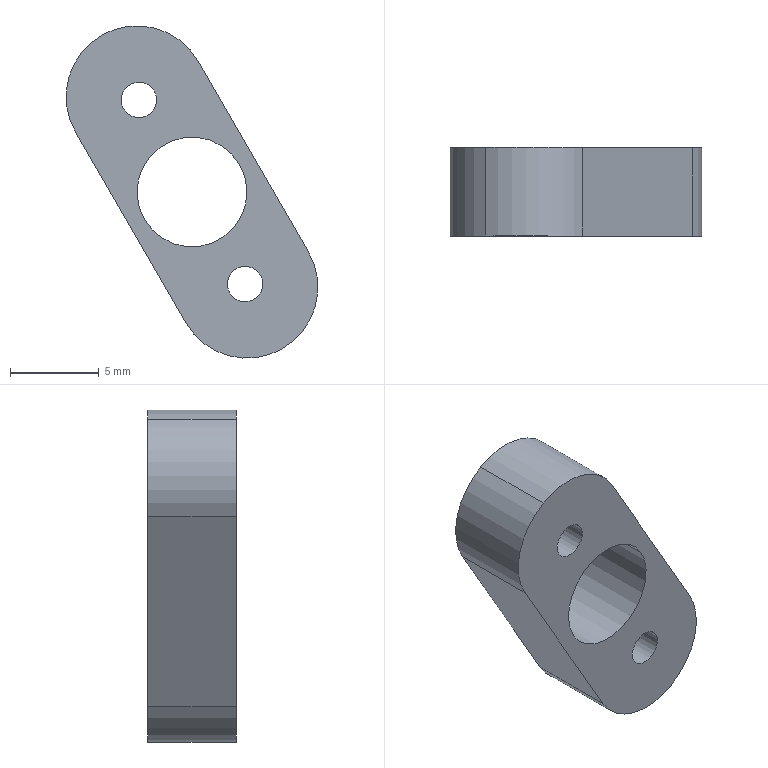Component | SolidWorks | WireConnectorBlock1-1 | 1 solid | 20 faces | box 14.21 x 5 x 18.76 mm | volume 566 mm3 | cylinder 10 | cone 6 | plane 4 | commonest cylinder face diameters 2 x4 8 x4 6.2 x2
STEP:
#1=COLOUR_RGB('',0.7922,0.8196,0.9333);
#2=FILL_AREA_STYLE_COLOUR('',#1);
#3=FILL_AREA_STYLE('',(#2));
#4=SURFACE_STYLE_FILL_AREA(#3);
#5=SURFACE_SIDE_STYLE('',(#4));
#6=SURFACE_STYLE_USAGE(.BOTH.,#5);
#7=PRESENTATION_STYLE_ASSIGNMENT((#6));
#8=CARTESIAN_POINT('',(1.551,0.8034,7.058));
#9=VERTEX_POINT('',#8);
#10=CARTESIAN_POINT('',(1.62,0.8034,7.097));
#11=VERTEX_POINT('',#10);
#12=CARTESIAN_POINT('',(1.585,0.8034,7.078));
#13=DIRECTION('',(0.,1.,0.));
#14=DIRECTION('',(0.866,0.,0.5));
#15=AXIS2_PLACEMENT_3D('',#12,#13,#14);
#16=CIRCLE('',#15,0.03937);
#17=EDGE_CURVE('',#9,#11,#16,.T.);
#18=ORIENTED_EDGE('',*,*,#17,.F.);
#19=CARTESIAN_POINT('',(1.548,0.8073,7.056));
#20=VERTEX_POINT('',#19);
#21=CARTESIAN_POINT('',(1.551,0.8034,7.058));
#22=DIRECTION('',(-0.6124,0.7071,-0.3536));
#23=VECTOR('',#22,39.37);
#24=LINE('',#21,#23);
#25=EDGE_CURVE('',#9,#20,#24,.T.);
#26=ORIENTED_EDGE('',*,*,#25,.T.);
#27=CARTESIAN_POINT('',(1.623,0.8073,7.099));
#28=VERTEX_POINT('',#27);
#29=CARTESIAN_POINT('',(1.585,0.8073,7.078));
#30=DIRECTION('',(0.,-1.,0.));
#31=DIRECTION('',(0.866,0.,0.5));
#32=AXIS2_PLACEMENT_3D('',#29,#30,#31);
#33=CIRCLE('',#32,0.04331);
#34=EDGE_CURVE('',#28,#20,#33,.T.);
#35=ORIENTED_EDGE('',*,*,#34,.F.);
#36=CARTESIAN_POINT('',(1.62,0.8034,7.097));
#37=DIRECTION('',(0.6124,0.7071,0.3536));
#38=VECTOR('',#37,39.37);
#39=LINE('',#36,#38);
#40=EDGE_CURVE('',#11,#28,#39,.T.);
#41=ORIENTED_EDGE('',*,*,#40,.F.);
#42=EDGE_LOOP('',(#18,#26,#35,#41));
#43=FACE_OUTER_BOUND('',#42,.T.);
#44=CARTESIAN_POINT('',(1.585,0.8034,7.078));
#45=DIRECTION('',(0.,1.,0.));
#46=DIRECTION('',(0.866,0.,0.5));
#47=AXIS2_PLACEMENT_3D('',#44,#45,#46);
#48=CONICAL_SURFACE('',#47,0.03937,0.7854);
#49=ADVANCED_FACE('',(#43),#48,.F.);
#50=CARTESIAN_POINT('',(1.362,0.8034,7.221));
#51=VERTEX_POINT('',#50);
#52=CARTESIAN_POINT('',(1.573,0.8034,7.343));
#53=VERTEX_POINT('',#52);
#54=CARTESIAN_POINT('',(1.467,0.8034,7.282));
#55=DIRECTION('',(0.,1.,0.));
#56=DIRECTION('',(0.866,0.,0.5));
#57=AXIS2_PLACEMENT_3D('',#54,#55,#56);
#58=CIRCLE('',#57,0.122);
#59=EDGE_CURVE('',#51,#53,#58,.T.);
#60=ORIENTED_EDGE('',*,*,#59,.F.);
#61=CARTESIAN_POINT('',(1.358,0.8073,7.219));
#62=VERTEX_POINT('',#61);
#63=CARTESIAN_POINT('',(1.362,0.8034,7.221));
#64=DIRECTION('',(-0.6124,0.7071,-0.3536));
#65=VECTOR('',#64,39.37);
#66=LINE('',#63,#65);
#67=EDGE_CURVE('',#51,#62,#66,.T.);
#68=ORIENTED_EDGE('',*,*,#67,.T.);
#69=CARTESIAN_POINT('',(1.576,0.8073,7.345));
#70=VERTEX_POINT('',#69);
#71=CARTESIAN_POINT('',(1.467,0.8073,7.282));
#72=DIRECTION('',(0.,-1.,0.));
#73=DIRECTION('',(0.866,0.,0.5));
#74=AXIS2_PLACEMENT_3D('',#71,#72,#73);
#75=CIRCLE('',#74,0.126);
#76=EDGE_CURVE('',#70,#62,#75,.T.);
#77=ORIENTED_EDGE('',*,*,#76,.F.);
#78=CARTESIAN_POINT('',(1.573,0.8034,7.343));
#79=DIRECTION('',(0.6124,0.7071,0.3536));
#80=VECTOR('',#79,39.37);
#81=LINE('',#78,#80);
#82=EDGE_CURVE('',#53,#70,#81,.T.);
#83=ORIENTED_EDGE('',*,*,#82,.F.);
#84=EDGE_LOOP('',(#60,#68,#77,#83));
#85=FACE_OUTER_BOUND('',#84,.T.);
#86=CARTESIAN_POINT('',(1.467,0.8034,7.282));
#87=DIRECTION('',(0.,1.,0.));
#88=DIRECTION('',(0.866,0.,0.5));
#89=AXIS2_PLACEMENT_3D('',#86,#87,#88);
#90=CONICAL_SURFACE('',#89,0.122,0.7854);
#91=ADVANCED_FACE('',(#85),#90,.F.);
#92=CARTESIAN_POINT('',(1.315,0.8034,7.467));
#93=VERTEX_POINT('',#92);
#94=CARTESIAN_POINT('',(1.383,0.8034,7.507));
#95=VERTEX_POINT('',#94);
#96=CARTESIAN_POINT('',(1.349,0.8034,7.487));
#97=DIRECTION('',(0.,1.,0.));
#98=DIRECTION('',(0.866,0.,0.5));
#99=AXIS2_PLACEMENT_3D('',#96,#97,#98);
#100=CIRCLE('',#99,0.03937);
#101=EDGE_CURVE('',#93,#95,#100,.T.);
#102=ORIENTED_EDGE('',*,*,#101,.F.);
#103=CARTESIAN_POINT('',(1.312,0.8073,7.465));
#104=VERTEX_POINT('',#103);
#105=CARTESIAN_POINT('',(1.315,0.8034,7.467));
#106=DIRECTION('',(-0.6124,0.7071,-0.3536));
#107=VECTOR('',#106,39.37);
#108=LINE('',#105,#107);
#109=EDGE_CURVE('',#93,#104,#108,.T.);
#110=ORIENTED_EDGE('',*,*,#109,.T.);
#111=CARTESIAN_POINT('',(1.387,0.8073,7.509));
#112=VERTEX_POINT('',#111);
#113=CARTESIAN_POINT('',(1.349,0.8073,7.487));
#114=DIRECTION('',(0.,-1.,0.));
#115=DIRECTION('',(0.866,0.,0.5));
#116=AXIS2_PLACEMENT_3D('',#113,#114,#115);
#117=CIRCLE('',#116,0.04331);
#118=EDGE_CURVE('',#112,#104,#117,.T.);
#119=ORIENTED_EDGE('',*,*,#118,.F.);
#120=CARTESIAN_POINT('',(1.383,0.8034,7.507));
#121=DIRECTION('',(0.6124,0.7071,0.3536));
#122=VECTOR('',#121,39.37);
#123=LINE('',#120,#122);
#124=EDGE_CURVE('',#95,#112,#123,.T.);
#125=ORIENTED_EDGE('',*,*,#124,.F.);
#126=EDGE_LOOP('',(#102,#110,#119,#125));
#127=FACE_OUTER_BOUND('',#126,.T.);
#128=CARTESIAN_POINT('',(1.349,0.8034,7.487));
#129=DIRECTION('',(0.,1.,0.));
#130=DIRECTION('',(0.866,0.,0.5));
#131=AXIS2_PLACEMENT_3D('',#128,#129,#130);
#132=CONICAL_SURFACE('',#131,0.03937,0.7854);
#133=ADVANCED_FACE('',(#127),#132,.F.);
#134=ORIENTED_EDGE('',*,*,#101,.T.);
#135=CARTESIAN_POINT('',(1.383,0.6105,7.507));
#136=VERTEX_POINT('',#135);
#137=CARTESIAN_POINT('',(1.383,0.8073,7.507));
#138=DIRECTION('',(0.,-1.,0.));
#139=VECTOR('',#138,39.37);
#140=LINE('',#137,#139);
#141=EDGE_CURVE('',#95,#136,#140,.T.);
#142=ORIENTED_EDGE('',*,*,#141,.T.);
#143=CARTESIAN_POINT('',(1.315,0.6105,7.467));
#144=VERTEX_POINT('',#143);
#145=CARTESIAN_POINT('',(1.349,0.6105,7.487));
#146=DIRECTION('',(0.,1.,0.));
#147=DIRECTION('',(-0.866,0.,-0.5));
#148=AXIS2_PLACEMENT_3D('',#145,#146,#147);
#149=CIRCLE('',#148,0.03937);
#150=EDGE_CURVE('',#144,#136,#149,.T.);
#151=ORIENTED_EDGE('',*,*,#150,.F.);
#152=CARTESIAN_POINT('',(1.315,0.8073,7.467));
#153=DIRECTION('',(0.,-1.,0.));
#154=VECTOR('',#153,39.37);
#155=LINE('',#152,#154);
#156=EDGE_CURVE('',#93,#144,#155,.T.);
#157=ORIENTED_EDGE('',*,*,#156,.F.);
#158=EDGE_LOOP('',(#134,#142,#151,#157));
#159=FACE_OUTER_BOUND('',#158,.T.);
#160=CARTESIAN_POINT('',(1.349,0.8073,7.487));
#161=DIRECTION('',(0.,-1.,0.));
#162=DIRECTION('',(-0.866,0.,-0.5));
#163=AXIS2_PLACEMENT_3D('',#160,#161,#162);
#164=CYLINDRICAL_SURFACE('',#163,0.03937);
#165=ADVANCED_FACE('',(#159),#164,.F.);
#166=ORIENTED_EDGE('',*,*,#17,.T.);
#167=CARTESIAN_POINT('',(1.62,0.6105,7.097));
#168=VERTEX_POINT('',#167);
#169=CARTESIAN_POINT('',(1.62,0.8073,7.097));
#170=DIRECTION('',(0.,-1.,0.));
#171=VECTOR('',#170,39.37);
#172=LINE('',#169,#171);
#173=EDGE_CURVE('',#11,#168,#172,.T.);
#174=ORIENTED_EDGE('',*,*,#173,.T.);
#175=CARTESIAN_POINT('',(1.551,0.6105,7.058));
#176=VERTEX_POINT('',#175);
#177=CARTESIAN_POINT('',(1.585,0.6105,7.078));
#178=DIRECTION('',(0.,1.,0.));
#179=DIRECTION('',(0.866,0.,0.5));
#180=AXIS2_PLACEMENT_3D('',#177,#178,#179);
#181=CIRCLE('',#180,0.03937);
#182=EDGE_CURVE('',#176,#168,#181,.T.);
#183=ORIENTED_EDGE('',*,*,#182,.F.);
#184=CARTESIAN_POINT('',(1.551,0.8073,7.058));
#185=DIRECTION('',(0.,-1.,0.));
#186=VECTOR('',#185,39.37);
#187=LINE('',#184,#186);
#188=EDGE_CURVE('',#9,#176,#187,.T.);
#189=ORIENTED_EDGE('',*,*,#188,.F.);
#190=EDGE_LOOP('',(#166,#174,#183,#189));
#191=FACE_OUTER_BOUND('',#190,.T.);
#192=CARTESIAN_POINT('',(1.585,0.8073,7.078));
#193=DIRECTION('',(0.,-1.,0.));
#194=DIRECTION('',(-0.866,0.,-0.5));
#195=AXIS2_PLACEMENT_3D('',#192,#193,#194);
#196=CYLINDRICAL_SURFACE('',#195,0.03937);
#197=ADVANCED_FACE('',(#191),#196,.F.);
#198=ORIENTED_EDGE('',*,*,#59,.T.);
#199=CARTESIAN_POINT('',(1.573,0.6105,7.343));
#200=VERTEX_POINT('',#199);
#201=CARTESIAN_POINT('',(1.573,0.8073,7.343));
#202=DIRECTION('',(0.,-1.,0.));
#203=VECTOR('',#202,39.37);
#204=LINE('',#201,#203);
#205=EDGE_CURVE('',#53,#200,#204,.T.);
#206=ORIENTED_EDGE('',*,*,#205,.T.);
#207=CARTESIAN_POINT('',(1.362,0.6105,7.221));
#208=VERTEX_POINT('',#207);
#209=CARTESIAN_POINT('',(1.467,0.6105,7.282));
#210=DIRECTION('',(0.,1.,0.));
#211=DIRECTION('',(0.866,0.,0.5));
#212=AXIS2_PLACEMENT_3D('',#209,#210,#211);
#213=CIRCLE('',#212,0.122);
#214=EDGE_CURVE('',#208,#200,#213,.T.);
#215=ORIENTED_EDGE('',*,*,#214,.F.);
#216=CARTESIAN_POINT('',(1.362,0.8073,7.221));
#217=DIRECTION('',(0.,-1.,0.));
#218=VECTOR('',#217,39.37);
#219=LINE('',#216,#218);
#220=EDGE_CURVE('',#51,#208,#219,.T.);
#221=ORIENTED_EDGE('',*,*,#220,.F.);
#222=EDGE_LOOP('',(#198,#206,#215,#221));
#223=FACE_OUTER_BOUND('',#222,.T.);
#224=CARTESIAN_POINT('',(1.467,0.8073,7.282));
#225=DIRECTION('',(0.,-1.,0.));
#226=DIRECTION('',(-0.866,0.,-0.5));
#227=AXIS2_PLACEMENT_3D('',#224,#225,#226);
#228=CYLINDRICAL_SURFACE('',#227,0.122);
#229=ADVANCED_FACE('',(#223),#228,.F.);
#230=ORIENTED_EDGE('',*,*,#118,.T.);
#231=CARTESIAN_POINT('',(1.349,0.8073,7.487));
#232=DIRECTION('',(0.,-1.,0.));
#233=DIRECTION('',(0.866,0.,0.5));
#234=AXIS2_PLACEMENT_3D('',#231,#232,#233);
#235=CIRCLE('',#234,0.04331);
#236=EDGE_CURVE('',#104,#112,#235,.T.);
#237=ORIENTED_EDGE('',*,*,#236,.T.);
#238=EDGE_LOOP('',(#230,#237));
#239=FACE_BOUND('',#238,.T.);
#240=ORIENTED_EDGE('',*,*,#76,.T.);
#241=CARTESIAN_POINT('',(1.467,0.8073,7.282));
#242=DIRECTION('',(0.,-1.,0.));
#243=DIRECTION('',(0.866,0.,0.5));
#244=AXIS2_PLACEMENT_3D('',#241,#242,#243);
#245=CIRCLE('',#244,0.126);
#246=EDGE_CURVE('',#62,#70,#245,.T.);
#247=ORIENTED_EDGE('',*,*,#246,.T.);
#248=EDGE_LOOP('',(#240,#247));
#249=FACE_BOUND('',#248,.T.);
#250=ORIENTED_EDGE('',*,*,#34,.T.);
#251=CARTESIAN_POINT('',(1.585,0.8073,7.078));
#252=DIRECTION('',(0.,-1.,0.));
#253=DIRECTION('',(0.866,0.,0.5));
#254=AXIS2_PLACEMENT_3D('',#251,#252,#253);
#255=CIRCLE('',#254,0.04331);
#256=EDGE_CURVE('',#20,#28,#255,.T.);
#257=ORIENTED_EDGE('',*,*,#256,.T.);
#258=EDGE_LOOP('',(#250,#257));
#259=FACE_BOUND('',#258,.T.);
#260=CARTESIAN_POINT('',(1.453,0.8073,6.992));
#261=VERTEX_POINT('',#260);
#262=CARTESIAN_POINT('',(1.209,0.8073,7.415));
#263=VERTEX_POINT('',#262);
#264=CARTESIAN_POINT('',(1.13,0.8073,7.552));
#265=DIRECTION('',(-0.5,0.,0.866));
#266=VECTOR('',#265,39.37);
#267=LINE('',#264,#266);
#268=EDGE_CURVE('',#261,#263,#267,.T.);
#269=ORIENTED_EDGE('',*,*,#268,.T.);
#270=CARTESIAN_POINT('',(1.266,0.8073,7.631));
#271=VERTEX_POINT('',#270);
#272=CARTESIAN_POINT('',(1.345,0.8073,7.494));
#273=DIRECTION('',(0.,1.,0.));
#274=DIRECTION('',(0.866,0.,0.5));
#275=AXIS2_PLACEMENT_3D('',#272,#273,#274);
#276=CIRCLE('',#275,0.1575);
#277=EDGE_CURVE('',#263,#271,#276,.T.);
#278=ORIENTED_EDGE('',*,*,#277,.T.);
#279=CARTESIAN_POINT('',(1.481,0.8073,7.573));
#280=VERTEX_POINT('',#279);
#281=CARTESIAN_POINT('',(1.345,0.8073,7.494));
#282=DIRECTION('',(0.,1.,0.));
#283=DIRECTION('',(0.866,0.,0.5));
#284=AXIS2_PLACEMENT_3D('',#281,#282,#283);
#285=CIRCLE('',#284,0.1575);
#286=EDGE_CURVE('',#271,#280,#285,.T.);
#287=ORIENTED_EDGE('',*,*,#286,.T.);
#288=CARTESIAN_POINT('',(1.726,0.8073,7.149));
#289=VERTEX_POINT('',#288);
#290=CARTESIAN_POINT('',(1.403,0.8073,7.709));
#291=DIRECTION('',(0.5,0.,-0.866));
#292=VECTOR('',#291,39.37);
#293=LINE('',#290,#292);
#294=EDGE_CURVE('',#280,#289,#293,.T.);
#295=ORIENTED_EDGE('',*,*,#294,.T.);
#296=CARTESIAN_POINT('',(1.668,0.8073,6.934));
#297=VERTEX_POINT('',#296);
#298=CARTESIAN_POINT('',(1.59,0.8073,7.071));
#299=DIRECTION('',(0.,1.,0.));
#300=DIRECTION('',(0.866,0.,0.5));
#301=AXIS2_PLACEMENT_3D('',#298,#299,#300);
#302=CIRCLE('',#301,0.1575);
#303=EDGE_CURVE('',#289,#297,#302,.T.);
#304=ORIENTED_EDGE('',*,*,#303,.T.);
#305=CARTESIAN_POINT('',(1.59,0.8073,7.071));
#306=DIRECTION('',(0.,1.,0.));
#307=DIRECTION('',(0.866,0.,0.5));
#308=AXIS2_PLACEMENT_3D('',#305,#306,#307);
#309=CIRCLE('',#308,0.1575);
#310=EDGE_CURVE('',#297,#261,#309,.T.);
#311=ORIENTED_EDGE('',*,*,#310,.T.);
#312=EDGE_LOOP('',(#269,#278,#287,#295,#304,#311));
#313=FACE_OUTER_BOUND('',#312,.T.);
#314=CARTESIAN_POINT('',(1.467,0.8073,7.282));
#315=DIRECTION('',(0.,1.,0.));
#316=DIRECTION('',(0.866,0.,0.5));
#317=AXIS2_PLACEMENT_3D('',#314,#315,#316);
#318=PLANE('',#317);
#319=ADVANCED_FACE('',(#239,#249,#259,#313),#318,.T.);
#320=CARTESIAN_POINT('',(1.481,0.6105,7.573));
#321=VERTEX_POINT('',#320);
#322=CARTESIAN_POINT('',(1.266,0.6105,7.631));
#323=VERTEX_POINT('',#322);
#324=CARTESIAN_POINT('',(1.345,0.6105,7.494));
#325=DIRECTION('',(0.,-1.,0.));
#326=DIRECTION('',(0.866,0.,0.5));
#327=AXIS2_PLACEMENT_3D('',#324,#325,#326);
#328=CIRCLE('',#327,0.1575);
#329=EDGE_CURVE('',#321,#323,#328,.T.);
#330=ORIENTED_EDGE('',*,*,#329,.T.);
#331=CARTESIAN_POINT('',(1.209,0.6105,7.415));
#332=VERTEX_POINT('',#331);
#333=CARTESIAN_POINT('',(1.345,0.6105,7.494));
#334=DIRECTION('',(0.,-1.,0.));
#335=DIRECTION('',(0.866,0.,0.5));
#336=AXIS2_PLACEMENT_3D('',#333,#334,#335);
#337=CIRCLE('',#336,0.1575);
#338=EDGE_CURVE('',#323,#332,#337,.T.);
#339=ORIENTED_EDGE('',*,*,#338,.T.);
#340=CARTESIAN_POINT('',(1.453,0.6105,6.992));
#341=VERTEX_POINT('',#340);
#342=CARTESIAN_POINT('',(1.13,0.6105,7.552));
#343=DIRECTION('',(-0.5,0.,0.866));
#344=VECTOR('',#343,39.37);
#345=LINE('',#342,#344);
#346=EDGE_CURVE('',#341,#332,#345,.T.);
#347=ORIENTED_EDGE('',*,*,#346,.F.);
#348=CARTESIAN_POINT('',(1.668,0.6105,6.934));
#349=VERTEX_POINT('',#348);
#350=CARTESIAN_POINT('',(1.59,0.6105,7.071));
#351=DIRECTION('',(0.,-1.,0.));
#352=DIRECTION('',(0.866,0.,0.5));
#353=AXIS2_PLACEMENT_3D('',#350,#351,#352);
#354=CIRCLE('',#353,0.1575);
#355=EDGE_CURVE('',#341,#349,#354,.T.);
#356=ORIENTED_EDGE('',*,*,#355,.T.);
#357=CARTESIAN_POINT('',(1.726,0.6105,7.149));
#358=VERTEX_POINT('',#357);
#359=CARTESIAN_POINT('',(1.59,0.6105,7.071));
#360=DIRECTION('',(0.,-1.,0.));
#361=DIRECTION('',(0.866,0.,0.5));
#362=AXIS2_PLACEMENT_3D('',#359,#360,#361);
#363=CIRCLE('',#362,0.1575);
#364=EDGE_CURVE('',#349,#358,#363,.T.);
#365=ORIENTED_EDGE('',*,*,#364,.T.);
#366=CARTESIAN_POINT('',(1.403,0.6105,7.709));
#367=DIRECTION('',(0.5,0.,-0.866));
#368=VECTOR('',#367,39.37);
#369=LINE('',#366,#368);
#370=EDGE_CURVE('',#321,#358,#369,.T.);
#371=ORIENTED_EDGE('',*,*,#370,.F.);
#372=EDGE_LOOP('',(#330,#339,#347,#356,#365,#371));
#373=FACE_OUTER_BOUND('',#372,.T.);
#374=ORIENTED_EDGE('',*,*,#214,.T.);
#375=CARTESIAN_POINT('',(1.467,0.6105,7.282));
#376=DIRECTION('',(0.,1.,0.));
#377=DIRECTION('',(0.866,0.,0.5));
#378=AXIS2_PLACEMENT_3D('',#375,#376,#377);
#379=CIRCLE('',#378,0.122);
#380=EDGE_CURVE('',#200,#208,#379,.T.);
#381=ORIENTED_EDGE('',*,*,#380,.T.);
#382=EDGE_LOOP('',(#374,#381));
#383=FACE_BOUND('',#382,.T.);
#384=ORIENTED_EDGE('',*,*,#182,.T.);
#385=CARTESIAN_POINT('',(1.585,0.6105,7.078));
#386=DIRECTION('',(0.,1.,0.));
#387=DIRECTION('',(0.866,0.,0.5));
#388=AXIS2_PLACEMENT_3D('',#385,#386,#387);
#389=CIRCLE('',#388,0.03937);
#390=EDGE_CURVE('',#168,#176,#389,.T.);
#391=ORIENTED_EDGE('',*,*,#390,.T.);
#392=EDGE_LOOP('',(#384,#391));
#393=FACE_BOUND('',#392,.T.);
#394=ORIENTED_EDGE('',*,*,#150,.T.);
#395=CARTESIAN_POINT('',(1.349,0.6105,7.487));
#396=DIRECTION('',(0.,1.,0.));
#397=DIRECTION('',(-0.866,0.,-0.5));
#398=AXIS2_PLACEMENT_3D('',#395,#396,#397);
#399=CIRCLE('',#398,0.03937);
#400=EDGE_CURVE('',#136,#144,#399,.T.);
#401=ORIENTED_EDGE('',*,*,#400,.T.);
#402=EDGE_LOOP('',(#394,#401));
#403=FACE_BOUND('',#402,.T.);
#404=CARTESIAN_POINT('',(1.467,0.6105,7.282));
#405=DIRECTION('',(0.,1.,0.));
#406=DIRECTION('',(0.866,0.,0.5));
#407=AXIS2_PLACEMENT_3D('',#404,#405,#406);
#408=PLANE('',#407);
#409=ADVANCED_FACE('',(#373,#383,#393,#403),#408,.F.);
#410=ORIENTED_EDGE('',*,*,#346,.T.);
#411=CARTESIAN_POINT('',(1.209,0.8073,7.415));
#412=DIRECTION('',(0.,1.,0.));
#413=VECTOR('',#412,39.37);
#414=LINE('',#411,#413);
#415=EDGE_CURVE('',#332,#263,#414,.T.);
#416=ORIENTED_EDGE('',*,*,#415,.T.);
#417=ORIENTED_EDGE('',*,*,#268,.F.);
#418=CARTESIAN_POINT('',(1.453,0.8073,6.992));
#419=DIRECTION('',(0.,-1.,0.));
#420=VECTOR('',#419,39.37);
#421=LINE('',#418,#420);
#422=EDGE_CURVE('',#261,#341,#421,.T.);
#423=ORIENTED_EDGE('',*,*,#422,.T.);
#424=EDGE_LOOP('',(#410,#416,#417,#423));
#425=FACE_OUTER_BOUND('',#424,.T.);
#426=CARTESIAN_POINT('',(1.13,0.8073,7.552));
#427=DIRECTION('',(0.866,0.,0.5));
#428=DIRECTION('',(0.5,0.,-0.866));
#429=AXIS2_PLACEMENT_3D('',#426,#427,#428);
#430=PLANE('',#429);
#431=ADVANCED_FACE('',(#425),#430,.F.);
#432=ORIENTED_EDGE('',*,*,#294,.F.);
#433=CARTESIAN_POINT('',(1.481,0.8073,7.573));
#434=DIRECTION('',(0.,-1.,0.));
#435=VECTOR('',#434,39.37);
#436=LINE('',#433,#435);
#437=EDGE_CURVE('',#280,#321,#436,.T.);
#438=ORIENTED_EDGE('',*,*,#437,.T.);
#439=ORIENTED_EDGE('',*,*,#370,.T.);
#440=CARTESIAN_POINT('',(1.726,0.8073,7.149));
#441=DIRECTION('',(0.,1.,0.));
#442=VECTOR('',#441,39.37);
#443=LINE('',#440,#442);
#444=EDGE_CURVE('',#358,#289,#443,.T.);
#445=ORIENTED_EDGE('',*,*,#444,.T.);
#446=EDGE_LOOP('',(#432,#438,#439,#445));
#447=FACE_OUTER_BOUND('',#446,.T.);
#448=CARTESIAN_POINT('',(1.403,0.8073,7.709));
#449=DIRECTION('',(-0.866,0.,-0.5));
#450=DIRECTION('',(-0.5,0.,0.866));
#451=AXIS2_PLACEMENT_3D('',#448,#449,#450);
#452=PLANE('',#451);
#453=ADVANCED_FACE('',(#447),#452,.F.);
#454=ORIENTED_EDGE('',*,*,#205,.F.);
#455=CARTESIAN_POINT('',(1.467,0.8034,7.282));
#456=DIRECTION('',(0.,1.,0.));
#457=DIRECTION('',(0.866,0.,0.5));
#458=AXIS2_PLACEMENT_3D('',#455,#456,#457);
#459=CIRCLE('',#458,0.122);
#460=EDGE_CURVE('',#53,#51,#459,.T.);
#461=ORIENTED_EDGE('',*,*,#460,.T.);
#462=ORIENTED_EDGE('',*,*,#220,.T.);
#463=ORIENTED_EDGE('',*,*,#380,.F.);
#464=EDGE_LOOP('',(#454,#461,#462,#463));
#465=FACE_OUTER_BOUND('',#464,.T.);
#466=CARTESIAN_POINT('',(1.467,0.8073,7.282));
#467=DIRECTION('',(0.,-1.,0.));
#468=DIRECTION('',(-0.866,0.,-0.5));
#469=AXIS2_PLACEMENT_3D('',#466,#467,#468);
#470=CYLINDRICAL_SURFACE('',#469,0.122);
#471=ADVANCED_FACE('',(#465),#470,.F.);
#472=ORIENTED_EDGE('',*,*,#173,.F.);
#473=CARTESIAN_POINT('',(1.585,0.8034,7.078));
#474=DIRECTION('',(0.,1.,0.));
#475=DIRECTION('',(0.866,0.,0.5));
#476=AXIS2_PLACEMENT_3D('',#473,#474,#475);
#477=CIRCLE('',#476,0.03937);
#478=EDGE_CURVE('',#11,#9,#477,.T.);
#479=ORIENTED_EDGE('',*,*,#478,.T.);
#480=ORIENTED_EDGE('',*,*,#188,.T.);
#481=ORIENTED_EDGE('',*,*,#390,.F.);
#482=EDGE_LOOP('',(#472,#479,#480,#481));
#483=FACE_OUTER_BOUND('',#482,.T.);
#484=CARTESIAN_POINT('',(1.585,0.8073,7.078));
#485=DIRECTION('',(0.,-1.,0.));
#486=DIRECTION('',(-0.866,0.,-0.5));
#487=AXIS2_PLACEMENT_3D('',#484,#485,#486);
#488=CYLINDRICAL_SURFACE('',#487,0.03937);
#489=ADVANCED_FACE('',(#483),#488,.F.);
#490=ORIENTED_EDGE('',*,*,#141,.F.);
#491=CARTESIAN_POINT('',(1.349,0.8034,7.487));
#492=DIRECTION('',(0.,1.,0.));
#493=DIRECTION('',(0.866,0.,0.5));
#494=AXIS2_PLACEMENT_3D('',#491,#492,#493);
#495=CIRCLE('',#494,0.03937);
#496=EDGE_CURVE('',#95,#93,#495,.T.);
#497=ORIENTED_EDGE('',*,*,#496,.T.);
#498=ORIENTED_EDGE('',*,*,#156,.T.);
#499=ORIENTED_EDGE('',*,*,#400,.F.);
#500=EDGE_LOOP('',(#490,#497,#498,#499));
#501=FACE_OUTER_BOUND('',#500,.T.);
#502=CARTESIAN_POINT('',(1.349,0.8073,7.487));
#503=DIRECTION('',(0.,-1.,0.));
#504=DIRECTION('',(-0.866,0.,-0.5));
#505=AXIS2_PLACEMENT_3D('',#502,#503,#504);
#506=CYLINDRICAL_SURFACE('',#505,0.03937);
#507=ADVANCED_FACE('',(#501),#506,.F.);
#508=ORIENTED_EDGE('',*,*,#437,.F.);
#509=ORIENTED_EDGE('',*,*,#286,.F.);
#510=CARTESIAN_POINT('',(1.266,0.8073,7.631));
#511=DIRECTION('',(0.,1.,0.));
#512=VECTOR('',#511,39.37);
#513=LINE('',#510,#512);
#514=EDGE_CURVE('',#323,#271,#513,.T.);
#515=ORIENTED_EDGE('',*,*,#514,.F.);
#516=ORIENTED_EDGE('',*,*,#329,.F.);
#517=EDGE_LOOP('',(#508,#509,#515,#516));
#518=FACE_OUTER_BOUND('',#517,.T.);
#519=CARTESIAN_POINT('',(1.345,0.8073,7.494));
#520=DIRECTION('',(0.,-1.,0.));
#521=DIRECTION('',(-0.866,0.,-0.5));
#522=AXIS2_PLACEMENT_3D('',#519,#520,#521);
#523=CYLINDRICAL_SURFACE('',#522,0.1575);
#524=ADVANCED_FACE('',(#518),#523,.T.);
#525=ORIENTED_EDGE('',*,*,#277,.F.);
#526=ORIENTED_EDGE('',*,*,#415,.F.);
#527=ORIENTED_EDGE('',*,*,#338,.F.);
#528=ORIENTED_EDGE('',*,*,#514,.T.);
#529=EDGE_LOOP('',(#525,#526,#527,#528));
#530=FACE_OUTER_BOUND('',#529,.T.);
#531=CARTESIAN_POINT('',(1.345,0.8073,7.494));
#532=DIRECTION('',(0.,-1.,0.));
#533=DIRECTION('',(-0.866,0.,-0.5));
#534=AXIS2_PLACEMENT_3D('',#531,#532,#533);
#535=CYLINDRICAL_SURFACE('',#534,0.1575);
#536=ADVANCED_FACE('',(#530),#535,.T.);
#537=CARTESIAN_POINT('',(1.668,0.8073,6.934));
#538=DIRECTION('',(0.,-1.,0.));
#539=VECTOR('',#538,39.37);
#540=LINE('',#537,#539);
#541=EDGE_CURVE('',#297,#349,#540,.T.);
#542=ORIENTED_EDGE('',*,*,#541,.F.);
#543=ORIENTED_EDGE('',*,*,#303,.F.);
#544=ORIENTED_EDGE('',*,*,#444,.F.);
#545=ORIENTED_EDGE('',*,*,#364,.F.);
#546=EDGE_LOOP('',(#542,#543,#544,#545));
#547=FACE_OUTER_BOUND('',#546,.T.);
#548=CARTESIAN_POINT('',(1.59,0.8073,7.071));
#549=DIRECTION('',(0.,-1.,0.));
#550=DIRECTION('',(-0.866,0.,-0.5));
#551=AXIS2_PLACEMENT_3D('',#548,#549,#550);
#552=CYLINDRICAL_SURFACE('',#551,0.1575);
#553=ADVANCED_FACE('',(#547),#552,.T.);
#554=ORIENTED_EDGE('',*,*,#310,.F.);
#555=ORIENTED_EDGE('',*,*,#541,.T.);
#556=ORIENTED_EDGE('',*,*,#355,.F.);
#557=ORIENTED_EDGE('',*,*,#422,.F.);
#558=EDGE_LOOP('',(#554,#555,#556,#557));
#559=FACE_OUTER_BOUND('',#558,.T.);
#560=CARTESIAN_POINT('',(1.59,0.8073,7.071));
#561=DIRECTION('',(0.,-1.,0.));
#562=DIRECTION('',(-0.866,0.,-0.5));
#563=AXIS2_PLACEMENT_3D('',#560,#561,#562);
#564=CYLINDRICAL_SURFACE('',#563,0.1575);
#565=ADVANCED_FACE('',(#559),#564,.T.);
#566=ORIENTED_EDGE('',*,*,#109,.F.);
#567=ORIENTED_EDGE('',*,*,#496,.F.);
#568=ORIENTED_EDGE('',*,*,#124,.T.);
#569=ORIENTED_EDGE('',*,*,#236,.F.);
#570=EDGE_LOOP('',(#566,#567,#568,#569));
#571=FACE_OUTER_BOUND('',#570,.T.);
#572=CARTESIAN_POINT('',(1.349,0.8034,7.487));
#573=DIRECTION('',(0.,1.,0.));
#574=DIRECTION('',(0.866,0.,0.5));
#575=AXIS2_PLACEMENT_3D('',#572,#573,#574);
#576=CONICAL_SURFACE('',#575,0.03937,0.7854);
#577=ADVANCED_FACE('',(#571),#576,.F.);
#578=ORIENTED_EDGE('',*,*,#67,.F.);
#579=ORIENTED_EDGE('',*,*,#460,.F.);
#580=ORIENTED_EDGE('',*,*,#82,.T.);
#581=ORIENTED_EDGE('',*,*,#246,.F.);
#582=EDGE_LOOP('',(#578,#579,#580,#581));
#583=FACE_OUTER_BOUND('',#582,.T.);
#584=CARTESIAN_POINT('',(1.467,0.8034,7.282));
#585=DIRECTION('',(0.,1.,0.));
#586=DIRECTION('',(0.866,0.,0.5));
#587=AXIS2_PLACEMENT_3D('',#584,#585,#586);
#588=CONICAL_SURFACE('',#587,0.122,0.7854);
#589=ADVANCED_FACE('',(#583),#588,.F.);
#590=ORIENTED_EDGE('',*,*,#25,.F.);
#591=ORIENTED_EDGE('',*,*,#478,.F.);
#592=ORIENTED_EDGE('',*,*,#40,.T.);
#593=ORIENTED_EDGE('',*,*,#256,.F.);
#594=EDGE_LOOP('',(#590,#591,#592,#593));
#595=FACE_OUTER_BOUND('',#594,.T.);
#596=CARTESIAN_POINT('',(1.585,0.8034,7.078));
#597=DIRECTION('',(0.,1.,0.));
#598=DIRECTION('',(0.866,0.,0.5));
#599=AXIS2_PLACEMENT_3D('',#596,#597,#598);
#600=CONICAL_SURFACE('',#599,0.03937,0.7854);
#601=ADVANCED_FACE('',(#595),#600,.F.);
#602=CLOSED_SHELL('',(#49,#91,#133,#165,#197,#229,#319,#409,#431,#453,#471,#489,#507,#524,#536,#553,#565,#577,#589,#601));
#603=MANIFOLD_SOLID_BREP('',#602);
#604=STYLED_ITEM('',(#7),#603);
#605=(LENGTH_UNIT()NAMED_UNIT(*)SI_UNIT($,.METRE.));
#606=LENGTH_MEASURE_WITH_UNIT(LENGTH_MEASURE(0.0254),#605);
#607=DIMENSIONAL_EXPONENTS(1.,0.,0.,0.,0.,0.,0.);
#608=(CONVERSION_BASED_UNIT('',#606)LENGTH_UNIT()NAMED_UNIT(#607));
#609=UNCERTAINTY_MEASURE_WITH_UNIT(LENGTH_MEASURE(0.00001),#608,'','');
#610=(NAMED_UNIT(*)PLANE_ANGLE_UNIT()SI_UNIT($,.RADIAN.));
#611=(NAMED_UNIT(*)SI_UNIT($,.STERADIAN.)SOLID_ANGLE_UNIT());
#612=(GEOMETRIC_REPRESENTATION_CONTEXT(3)GLOBAL_UNCERTAINTY_ASSIGNED_CONTEXT((#609))GLOBAL_UNIT_ASSIGNED_CONTEXT((#608,#610,#611))REPRESENTATION_CONTEXT('',''));
#613=MECHANICAL_DESIGN_GEOMETRIC_PRESENTATION_REPRESENTATION('',(#604),#612);
#614=PRESENTATION_LAYER_ASSIGNMENT('','',(#604));
#615=CARTESIAN_POINT('',(0.,0.,0.));
#616=DIRECTION('',(0.,0.,1.));
#617=DIRECTION('',(1.,0.,0.));
#618=AXIS2_PLACEMENT_3D('',#615,#616,#617);
#619=(LENGTH_UNIT()NAMED_UNIT(*)SI_UNIT($,.METRE.));
#620=LENGTH_MEASURE_WITH_UNIT(LENGTH_MEASURE(0.0254),#619);
#621=DIMENSIONAL_EXPONENTS(1.,0.,0.,0.,0.,0.,0.);
#622=(CONVERSION_BASED_UNIT('',#620)LENGTH_UNIT()NAMED_UNIT(#621));
#623=UNCERTAINTY_MEASURE_WITH_UNIT(LENGTH_MEASURE(0.00001),#622,'','');
#624=(NAMED_UNIT(*)PLANE_ANGLE_UNIT()SI_UNIT($,.RADIAN.));
#625=(NAMED_UNIT(*)SI_UNIT($,.STERADIAN.)SOLID_ANGLE_UNIT());
#626=(GEOMETRIC_REPRESENTATION_CONTEXT(3)GLOBAL_UNCERTAINTY_ASSIGNED_CONTEXT((#623))GLOBAL_UNIT_ASSIGNED_CONTEXT((#622,#624,#625))REPRESENTATION_CONTEXT('',''));
#627=ADVANCED_BREP_SHAPE_REPRESENTATION('',(#603,#618),#626);